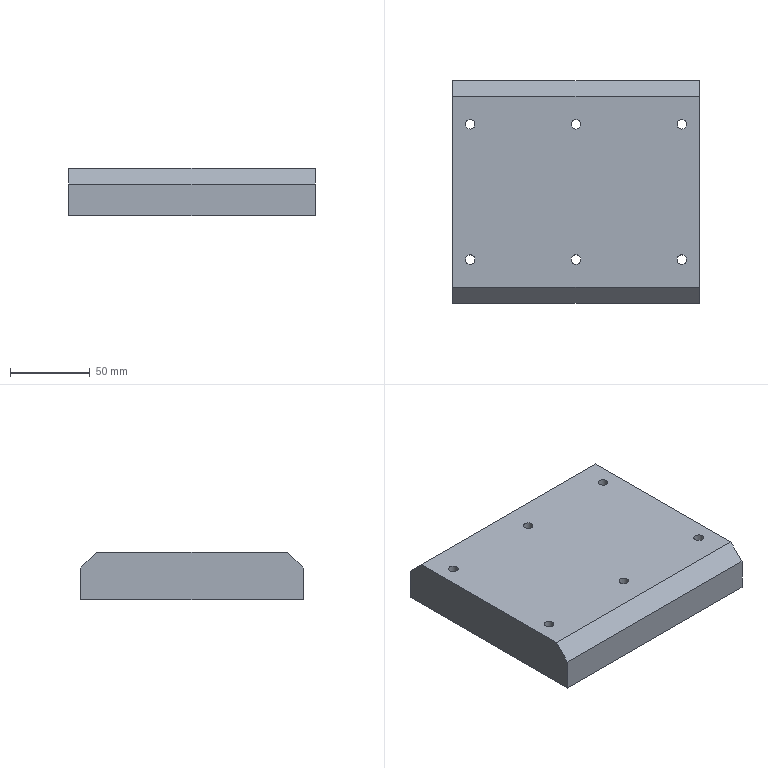Component | NX | 24__27 | 1 solid | 26 faces | volume 622871 mm3 | plane 14 | cylinder 12 | commonest cylinder face diameters 6 x6 14 x6